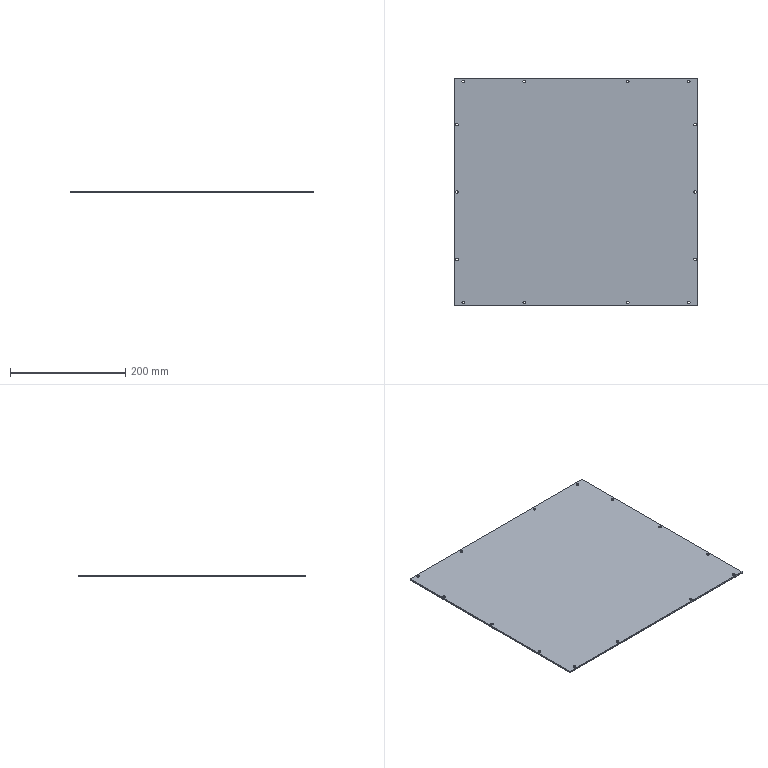CAM job | Mastercam | mm | 4 operations | part box 423.6 x 393.6 x 3
1. Contour (Ramp) | 10 - 10 平铣刀
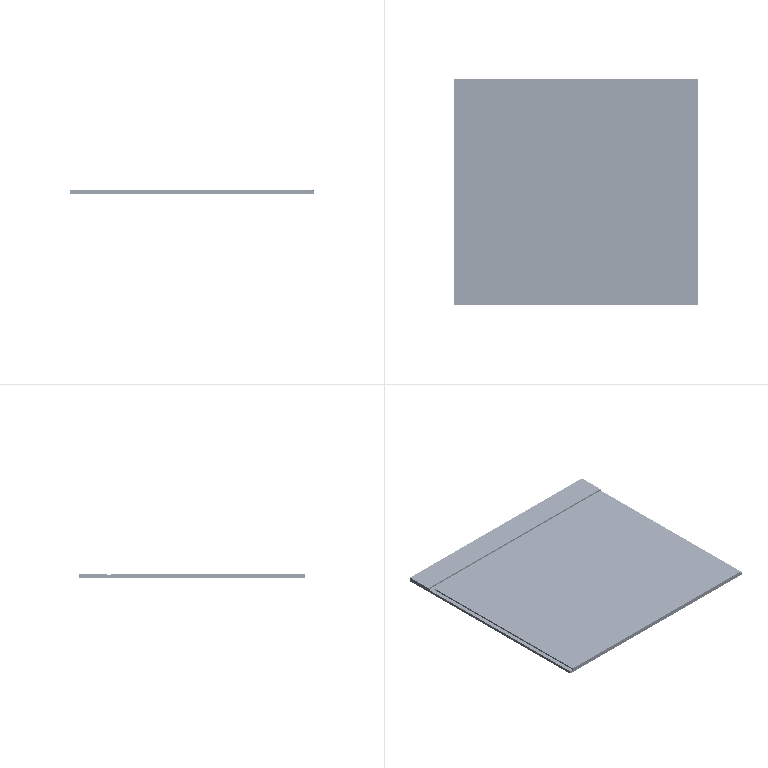2. Contour (2D) | 10 - 10 平铣刀
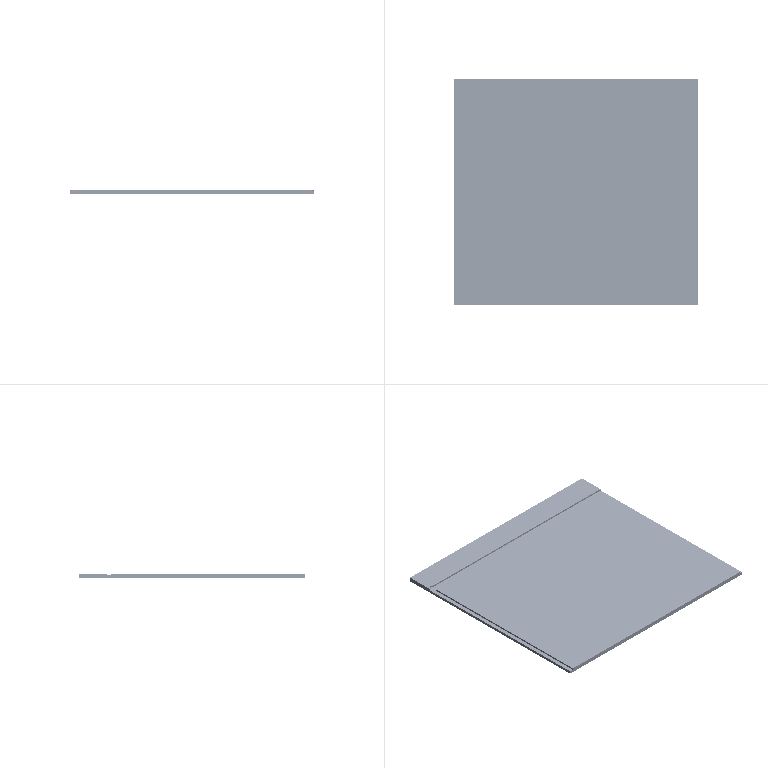3. Drill/Counterbore | 7 - 4 倒角刀
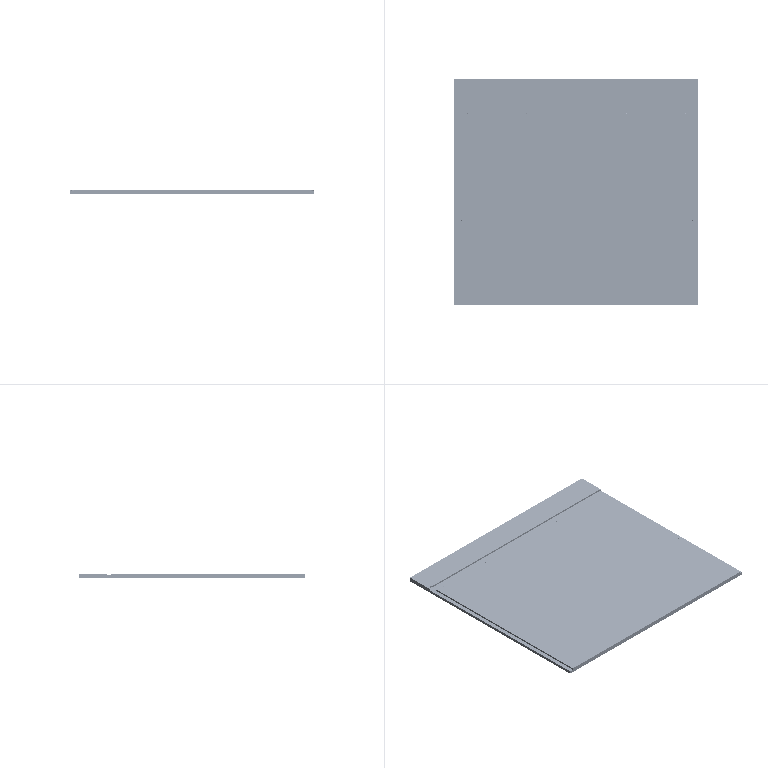4. Contour (2D chamfer) | 7 - 4 倒角刀